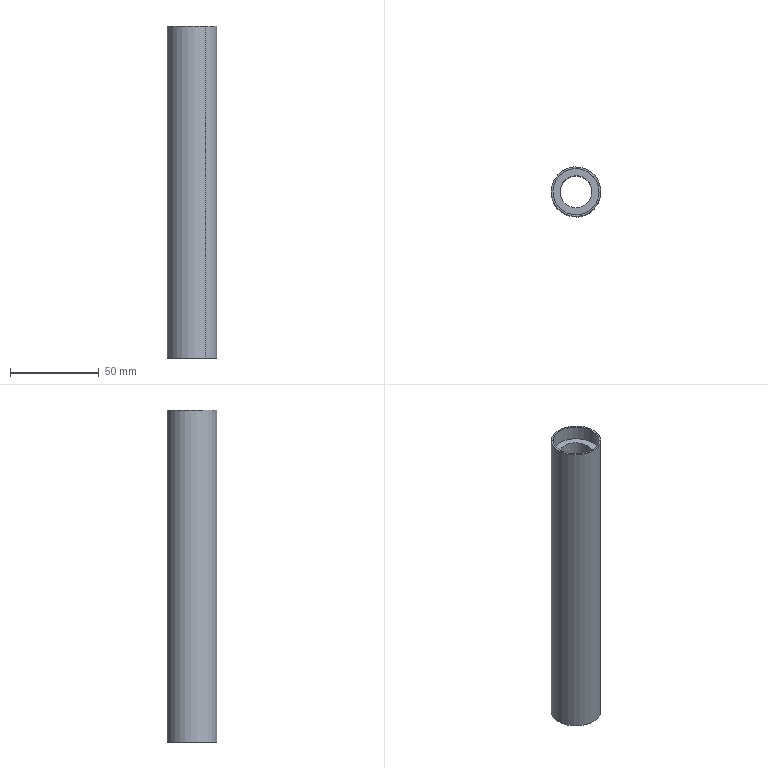Component | SolidWorks | Roller2-1 | 1 solid | 12 faces | box 28 x 28 x 187 mm | volume 63137 mm3 | cylinder 8 | plane 4 | commonest cylinder face diameters 26 x4 18 x2 28 x2
build123d program:
from build123d import *

# Parameters (mm, degrees)
MOVE_FACE1_BY = 1


with BuildPart() as part:
    # Sketch1 → Revolve1 (revolve)
    with BuildSketch(Plane(origin=(0, 0, 0), x_dir=(-1, 0, 0), z_dir=(0, 0, -1)), mode=Mode.PRIVATE) as revolve1_sk:
        Polygon((-85.5, 13), (-85.5, 9), (85.5, 9), (85.5, 13), (93.5, 13), (93.5, 15), (-93.5, 15), (-93.5, 13), align=None)
    revolve(revolve1_sk.sketch.rotate(Axis((93.5, 0, 0), (-1, 0, 0)), 270), axis=Axis((93.5, 0, 0), (-1, 0, 0)))

    # Move Face1: a curved face moved inward by 1.0
    add(Solid.thicken(part.faces().sort_by_distance((0, 0, -15))[0], -MOVE_FACE1_BY), mode=Mode.SUBTRACT)


solid = part.part

# Placed as in the assembly
solid = solid.moved(Location((-66, -158, -96.5), (0, 90, 0)))
STEP:
#1=COLOUR_RGB('',0.7922,0.8196,0.9333);
#2=FILL_AREA_STYLE_COLOUR('',#1);
#3=FILL_AREA_STYLE('',(#2));
#4=SURFACE_STYLE_FILL_AREA(#3);
#5=SURFACE_SIDE_STYLE('',(#4));
#6=SURFACE_STYLE_USAGE(.BOTH.,#5);
#7=PRESENTATION_STYLE_ASSIGNMENT((#6));
#8=CARTESIAN_POINT('',(-2.407,-6.519,-0.4331));
#9=VERTEX_POINT('',#8);
#10=CARTESIAN_POINT('',(-2.79,-5.922,-0.4331));
#11=VERTEX_POINT('',#10);
#12=CARTESIAN_POINT('',(-2.598,-6.22,-0.4331));
#13=DIRECTION('',(-0.,0.,-1.));
#14=DIRECTION('',(-0.5401,0.8416,0.));
#15=AXIS2_PLACEMENT_3D('',#12,#13,#14);
#16=CIRCLE('',#15,0.3543);
#17=EDGE_CURVE('',#9,#11,#16,.T.);
#18=ORIENTED_EDGE('',*,*,#17,.F.);
#19=CARTESIAN_POINT('',(-2.407,-6.519,-7.165));
#20=VERTEX_POINT('',#19);
#21=CARTESIAN_POINT('',(-2.407,-6.519,-0.1181));
#22=DIRECTION('',(-0.,0.,-1.));
#23=VECTOR('',#22,39.37);
#24=LINE('',#21,#23);
#25=EDGE_CURVE('',#9,#20,#24,.T.);
#26=ORIENTED_EDGE('',*,*,#25,.T.);
#27=CARTESIAN_POINT('',(-2.79,-5.922,-7.165));
#28=VERTEX_POINT('',#27);
#29=CARTESIAN_POINT('',(-2.598,-6.22,-7.165));
#30=DIRECTION('',(-0.,0.,-1.));
#31=DIRECTION('',(-0.5401,0.8416,0.));
#32=AXIS2_PLACEMENT_3D('',#29,#30,#31);
#33=CIRCLE('',#32,0.3543);
#34=EDGE_CURVE('',#20,#28,#33,.T.);
#35=ORIENTED_EDGE('',*,*,#34,.T.);
#36=CARTESIAN_POINT('',(-2.79,-5.922,-0.1181));
#37=DIRECTION('',(-0.,0.,-1.));
#38=VECTOR('',#37,39.37);
#39=LINE('',#36,#38);
#40=EDGE_CURVE('',#11,#28,#39,.T.);
#41=ORIENTED_EDGE('',*,*,#40,.F.);
#42=EDGE_LOOP('',(#18,#26,#35,#41));
#43=FACE_OUTER_BOUND('',#42,.T.);
#44=CARTESIAN_POINT('',(-2.598,-6.22,-0.1181));
#45=DIRECTION('',(-0.,0.,-1.));
#46=DIRECTION('',(-0.5401,0.8416,0.));
#47=AXIS2_PLACEMENT_3D('',#44,#45,#46);
#48=CYLINDRICAL_SURFACE('',#47,0.3543);
#49=ADVANCED_FACE('',(#43),#48,.F.);
#50=CARTESIAN_POINT('',(-2.322,-6.651,-7.165));
#51=VERTEX_POINT('',#50);
#52=CARTESIAN_POINT('',(-2.875,-5.79,-7.165));
#53=VERTEX_POINT('',#52);
#54=CARTESIAN_POINT('',(-2.598,-6.22,-7.165));
#55=DIRECTION('',(-0.,0.,-1.));
#56=DIRECTION('',(-0.5401,0.8416,0.));
#57=AXIS2_PLACEMENT_3D('',#54,#55,#56);
#58=CIRCLE('',#57,0.5118);
#59=EDGE_CURVE('',#51,#53,#58,.T.);
#60=ORIENTED_EDGE('',*,*,#59,.F.);
#61=CARTESIAN_POINT('',(-2.322,-6.651,-7.48));
#62=VERTEX_POINT('',#61);
#63=CARTESIAN_POINT('',(-2.322,-6.651,-0.1181));
#64=DIRECTION('',(-0.,0.,-1.));
#65=VECTOR('',#64,39.37);
#66=LINE('',#63,#65);
#67=EDGE_CURVE('',#51,#62,#66,.T.);
#68=ORIENTED_EDGE('',*,*,#67,.T.);
#69=CARTESIAN_POINT('',(-2.875,-5.79,-7.48));
#70=VERTEX_POINT('',#69);
#71=CARTESIAN_POINT('',(-2.598,-6.22,-7.48));
#72=DIRECTION('',(-0.,0.,-1.));
#73=DIRECTION('',(-0.5401,0.8416,0.));
#74=AXIS2_PLACEMENT_3D('',#71,#72,#73);
#75=CIRCLE('',#74,0.5118);
#76=EDGE_CURVE('',#62,#70,#75,.T.);
#77=ORIENTED_EDGE('',*,*,#76,.T.);
#78=CARTESIAN_POINT('',(-2.875,-5.79,-0.1181));
#79=DIRECTION('',(-0.,0.,-1.));
#80=VECTOR('',#79,39.37);
#81=LINE('',#78,#80);
#82=EDGE_CURVE('',#53,#70,#81,.T.);
#83=ORIENTED_EDGE('',*,*,#82,.F.);
#84=EDGE_LOOP('',(#60,#68,#77,#83));
#85=FACE_OUTER_BOUND('',#84,.T.);
#86=CARTESIAN_POINT('',(-2.598,-6.22,-0.1181));
#87=DIRECTION('',(-0.,0.,-1.));
#88=DIRECTION('',(-0.5401,0.8416,0.));
#89=AXIS2_PLACEMENT_3D('',#86,#87,#88);
#90=CYLINDRICAL_SURFACE('',#89,0.5118);
#91=ADVANCED_FACE('',(#85),#90,.F.);
#92=CARTESIAN_POINT('',(-2.896,-5.757,-0.1181));
#93=VERTEX_POINT('',#92);
#94=CARTESIAN_POINT('',(-2.301,-6.684,-0.1181));
#95=VERTEX_POINT('',#94);
#96=CARTESIAN_POINT('',(-2.598,-6.22,-0.1181));
#97=DIRECTION('',(-0.,0.,-1.));
#98=DIRECTION('',(0.5401,-0.8416,-0.));
#99=AXIS2_PLACEMENT_3D('',#96,#97,#98);
#100=CIRCLE('',#99,0.5512);
#101=EDGE_CURVE('',#93,#95,#100,.T.);
#102=ORIENTED_EDGE('',*,*,#101,.T.);
#103=CARTESIAN_POINT('',(-2.301,-6.684,-7.48));
#104=VERTEX_POINT('',#103);
#105=CARTESIAN_POINT('',(-2.301,-6.684,-0.1181));
#106=DIRECTION('',(-0.,0.,-1.));
#107=VECTOR('',#106,39.37);
#108=LINE('',#105,#107);
#109=EDGE_CURVE('',#95,#104,#108,.T.);
#110=ORIENTED_EDGE('',*,*,#109,.T.);
#111=CARTESIAN_POINT('',(-2.896,-5.757,-7.48));
#112=VERTEX_POINT('',#111);
#113=CARTESIAN_POINT('',(-2.598,-6.22,-7.48));
#114=DIRECTION('',(-0.,0.,-1.));
#115=DIRECTION('',(-0.5401,0.8416,0.));
#116=AXIS2_PLACEMENT_3D('',#113,#114,#115);
#117=CIRCLE('',#116,0.5512);
#118=EDGE_CURVE('',#112,#104,#117,.T.);
#119=ORIENTED_EDGE('',*,*,#118,.F.);
#120=CARTESIAN_POINT('',(-2.896,-5.757,-0.1181));
#121=DIRECTION('',(-0.,0.,-1.));
#122=VECTOR('',#121,39.37);
#123=LINE('',#120,#122);
#124=EDGE_CURVE('',#93,#112,#123,.T.);
#125=ORIENTED_EDGE('',*,*,#124,.F.);
#126=EDGE_LOOP('',(#102,#110,#119,#125));
#127=FACE_OUTER_BOUND('',#126,.T.);
#128=CARTESIAN_POINT('',(-2.598,-6.22,-0.1181));
#129=DIRECTION('',(-0.,0.,-1.));
#130=DIRECTION('',(-0.5401,0.8416,0.));
#131=AXIS2_PLACEMENT_3D('',#128,#129,#130);
#132=CYLINDRICAL_SURFACE('',#131,0.5512);
#133=ADVANCED_FACE('',(#127),#132,.T.);
#134=CARTESIAN_POINT('',(-2.322,-6.651,-0.1181));
#135=VERTEX_POINT('',#134);
#136=CARTESIAN_POINT('',(-2.875,-5.79,-0.1181));
#137=VERTEX_POINT('',#136);
#138=CARTESIAN_POINT('',(-2.598,-6.22,-0.1181));
#139=DIRECTION('',(-0.,0.,-1.));
#140=DIRECTION('',(-0.5401,0.8416,0.));
#141=AXIS2_PLACEMENT_3D('',#138,#139,#140);
#142=CIRCLE('',#141,0.5118);
#143=EDGE_CURVE('',#135,#137,#142,.T.);
#144=ORIENTED_EDGE('',*,*,#143,.F.);
#145=CARTESIAN_POINT('',(-2.322,-6.651,-0.4331));
#146=VERTEX_POINT('',#145);
#147=CARTESIAN_POINT('',(-2.322,-6.651,-0.1181));
#148=DIRECTION('',(-0.,0.,-1.));
#149=VECTOR('',#148,39.37);
#150=LINE('',#147,#149);
#151=EDGE_CURVE('',#135,#146,#150,.T.);
#152=ORIENTED_EDGE('',*,*,#151,.T.);
#153=CARTESIAN_POINT('',(-2.875,-5.79,-0.4331));
#154=VERTEX_POINT('',#153);
#155=CARTESIAN_POINT('',(-2.598,-6.22,-0.4331));
#156=DIRECTION('',(-0.,0.,-1.));
#157=DIRECTION('',(-0.5401,0.8416,0.));
#158=AXIS2_PLACEMENT_3D('',#155,#156,#157);
#159=CIRCLE('',#158,0.5118);
#160=EDGE_CURVE('',#146,#154,#159,.T.);
#161=ORIENTED_EDGE('',*,*,#160,.T.);
#162=CARTESIAN_POINT('',(-2.875,-5.79,-0.1181));
#163=DIRECTION('',(-0.,0.,-1.));
#164=VECTOR('',#163,39.37);
#165=LINE('',#162,#164);
#166=EDGE_CURVE('',#137,#154,#165,.T.);
#167=ORIENTED_EDGE('',*,*,#166,.F.);
#168=EDGE_LOOP('',(#144,#152,#161,#167));
#169=FACE_OUTER_BOUND('',#168,.T.);
#170=CARTESIAN_POINT('',(-2.598,-6.22,-0.1181));
#171=DIRECTION('',(-0.,0.,-1.));
#172=DIRECTION('',(-0.5401,0.8416,0.));
#173=AXIS2_PLACEMENT_3D('',#170,#171,#172);
#174=CYLINDRICAL_SURFACE('',#173,0.5118);
#175=ADVANCED_FACE('',(#169),#174,.F.);
#176=ORIENTED_EDGE('',*,*,#151,.F.);
#177=CARTESIAN_POINT('',(-2.598,-6.22,-0.1181));
#178=DIRECTION('',(-0.,0.,-1.));
#179=DIRECTION('',(-0.5401,0.8416,0.));
#180=AXIS2_PLACEMENT_3D('',#177,#178,#179);
#181=CIRCLE('',#180,0.5118);
#182=EDGE_CURVE('',#137,#135,#181,.T.);
#183=ORIENTED_EDGE('',*,*,#182,.F.);
#184=ORIENTED_EDGE('',*,*,#166,.T.);
#185=CARTESIAN_POINT('',(-2.598,-6.22,-0.4331));
#186=DIRECTION('',(-0.,0.,-1.));
#187=DIRECTION('',(-0.5401,0.8416,0.));
#188=AXIS2_PLACEMENT_3D('',#185,#186,#187);
#189=CIRCLE('',#188,0.5118);
#190=EDGE_CURVE('',#154,#146,#189,.T.);
#191=ORIENTED_EDGE('',*,*,#190,.T.);
#192=EDGE_LOOP('',(#176,#183,#184,#191));
#193=FACE_OUTER_BOUND('',#192,.T.);
#194=CARTESIAN_POINT('',(-2.598,-6.22,-0.1181));
#195=DIRECTION('',(-0.,0.,-1.));
#196=DIRECTION('',(-0.5401,0.8416,0.));
#197=AXIS2_PLACEMENT_3D('',#194,#195,#196);
#198=CYLINDRICAL_SURFACE('',#197,0.5118);
#199=ADVANCED_FACE('',(#193),#198,.F.);
#200=ORIENTED_EDGE('',*,*,#182,.T.);
#201=ORIENTED_EDGE('',*,*,#143,.T.);
#202=EDGE_LOOP('',(#200,#201));
#203=FACE_BOUND('',#202,.T.);
#204=ORIENTED_EDGE('',*,*,#101,.F.);
#205=CARTESIAN_POINT('',(-2.598,-6.22,-0.1181));
#206=DIRECTION('',(-0.,0.,-1.));
#207=DIRECTION('',(0.5401,-0.8416,-0.));
#208=AXIS2_PLACEMENT_3D('',#205,#206,#207);
#209=CIRCLE('',#208,0.5512);
#210=EDGE_CURVE('',#95,#93,#209,.T.);
#211=ORIENTED_EDGE('',*,*,#210,.F.);
#212=EDGE_LOOP('',(#204,#211));
#213=FACE_OUTER_BOUND('',#212,.T.);
#214=CARTESIAN_POINT('',(-2.101,-5.902,-0.1181));
#215=DIRECTION('',(0.,-0.,1.));
#216=DIRECTION('',(0.5401,-0.8416,-0.));
#217=AXIS2_PLACEMENT_3D('',#214,#215,#216);
#218=PLANE('',#217);
#219=ADVANCED_FACE('',(#203,#213),#218,.T.);
#220=ORIENTED_EDGE('',*,*,#109,.F.);
#221=ORIENTED_EDGE('',*,*,#210,.T.);
#222=ORIENTED_EDGE('',*,*,#124,.T.);
#223=CARTESIAN_POINT('',(-2.598,-6.22,-7.48));
#224=DIRECTION('',(-0.,0.,-1.));
#225=DIRECTION('',(-0.5401,0.8416,0.));
#226=AXIS2_PLACEMENT_3D('',#223,#224,#225);
#227=CIRCLE('',#226,0.5512);
#228=EDGE_CURVE('',#104,#112,#227,.T.);
#229=ORIENTED_EDGE('',*,*,#228,.F.);
#230=EDGE_LOOP('',(#220,#221,#222,#229));
#231=FACE_OUTER_BOUND('',#230,.T.);
#232=CARTESIAN_POINT('',(-2.598,-6.22,-0.1181));
#233=DIRECTION('',(-0.,0.,-1.));
#234=DIRECTION('',(-0.5401,0.8416,0.));
#235=AXIS2_PLACEMENT_3D('',#232,#233,#234);
#236=CYLINDRICAL_SURFACE('',#235,0.5512);
#237=ADVANCED_FACE('',(#231),#236,.T.);
#238=ORIENTED_EDGE('',*,*,#118,.T.);
#239=ORIENTED_EDGE('',*,*,#228,.T.);
#240=EDGE_LOOP('',(#238,#239));
#241=FACE_OUTER_BOUND('',#240,.T.);
#242=CARTESIAN_POINT('',(-2.598,-6.22,-7.48));
#243=DIRECTION('',(-0.,0.,-1.));
#244=DIRECTION('',(-0.5401,0.8416,0.));
#245=AXIS2_PLACEMENT_3D('',#242,#243,#244);
#246=CIRCLE('',#245,0.5118);
#247=EDGE_CURVE('',#70,#62,#246,.T.);
#248=ORIENTED_EDGE('',*,*,#247,.F.);
#249=ORIENTED_EDGE('',*,*,#76,.F.);
#250=EDGE_LOOP('',(#248,#249));
#251=FACE_BOUND('',#250,.T.);
#252=CARTESIAN_POINT('',(-2.168,-5.944,-7.48));
#253=DIRECTION('',(-0.,0.,-1.));
#254=DIRECTION('',(-0.5401,0.8416,0.));
#255=AXIS2_PLACEMENT_3D('',#252,#253,#254);
#256=PLANE('',#255);
#257=ADVANCED_FACE('',(#241,#251),#256,.T.);
#258=ORIENTED_EDGE('',*,*,#67,.F.);
#259=CARTESIAN_POINT('',(-2.598,-6.22,-7.165));
#260=DIRECTION('',(-0.,0.,-1.));
#261=DIRECTION('',(-0.5401,0.8416,0.));
#262=AXIS2_PLACEMENT_3D('',#259,#260,#261);
#263=CIRCLE('',#262,0.5118);
#264=EDGE_CURVE('',#53,#51,#263,.T.);
#265=ORIENTED_EDGE('',*,*,#264,.F.);
#266=ORIENTED_EDGE('',*,*,#82,.T.);
#267=ORIENTED_EDGE('',*,*,#247,.T.);
#268=EDGE_LOOP('',(#258,#265,#266,#267));
#269=FACE_OUTER_BOUND('',#268,.T.);
#270=CARTESIAN_POINT('',(-2.598,-6.22,-0.1181));
#271=DIRECTION('',(-0.,0.,-1.));
#272=DIRECTION('',(-0.5401,0.8416,0.));
#273=AXIS2_PLACEMENT_3D('',#270,#271,#272);
#274=CYLINDRICAL_SURFACE('',#273,0.5118);
#275=ADVANCED_FACE('',(#269),#274,.F.);
#276=ORIENTED_EDGE('',*,*,#264,.T.);
#277=ORIENTED_EDGE('',*,*,#59,.T.);
#278=EDGE_LOOP('',(#276,#277));
#279=FACE_OUTER_BOUND('',#278,.T.);
#280=CARTESIAN_POINT('',(-2.598,-6.22,-7.165));
#281=DIRECTION('',(-0.,0.,-1.));
#282=DIRECTION('',(-0.5401,0.8416,0.));
#283=AXIS2_PLACEMENT_3D('',#280,#281,#282);
#284=CIRCLE('',#283,0.3543);
#285=EDGE_CURVE('',#28,#20,#284,.T.);
#286=ORIENTED_EDGE('',*,*,#285,.F.);
#287=ORIENTED_EDGE('',*,*,#34,.F.);
#288=EDGE_LOOP('',(#286,#287));
#289=FACE_BOUND('',#288,.T.);
#290=CARTESIAN_POINT('',(-2.3,-6.029,-7.165));
#291=DIRECTION('',(-0.,0.,-1.));
#292=DIRECTION('',(-0.5401,0.8416,0.));
#293=AXIS2_PLACEMENT_3D('',#290,#291,#292);
#294=PLANE('',#293);
#295=ADVANCED_FACE('',(#279,#289),#294,.T.);
#296=ORIENTED_EDGE('',*,*,#25,.F.);
#297=CARTESIAN_POINT('',(-2.598,-6.22,-0.4331));
#298=DIRECTION('',(-0.,0.,-1.));
#299=DIRECTION('',(-0.5401,0.8416,0.));
#300=AXIS2_PLACEMENT_3D('',#297,#298,#299);
#301=CIRCLE('',#300,0.3543);
#302=EDGE_CURVE('',#11,#9,#301,.T.);
#303=ORIENTED_EDGE('',*,*,#302,.F.);
#304=ORIENTED_EDGE('',*,*,#40,.T.);
#305=ORIENTED_EDGE('',*,*,#285,.T.);
#306=EDGE_LOOP('',(#296,#303,#304,#305));
#307=FACE_OUTER_BOUND('',#306,.T.);
#308=CARTESIAN_POINT('',(-2.598,-6.22,-0.1181));
#309=DIRECTION('',(-0.,0.,-1.));
#310=DIRECTION('',(-0.5401,0.8416,0.));
#311=AXIS2_PLACEMENT_3D('',#308,#309,#310);
#312=CYLINDRICAL_SURFACE('',#311,0.3543);
#313=ADVANCED_FACE('',(#307),#312,.F.);
#314=ORIENTED_EDGE('',*,*,#302,.T.);
#315=ORIENTED_EDGE('',*,*,#17,.T.);
#316=EDGE_LOOP('',(#314,#315));
#317=FACE_BOUND('',#316,.T.);
#318=ORIENTED_EDGE('',*,*,#190,.F.);
#319=ORIENTED_EDGE('',*,*,#160,.F.);
#320=EDGE_LOOP('',(#318,#319));
#321=FACE_OUTER_BOUND('',#320,.T.);
#322=CARTESIAN_POINT('',(-2.168,-5.944,-0.4331));
#323=DIRECTION('',(0.,-0.,1.));
#324=DIRECTION('',(0.5401,-0.8416,-0.));
#325=AXIS2_PLACEMENT_3D('',#322,#323,#324);
#326=PLANE('',#325);
#327=ADVANCED_FACE('',(#317,#321),#326,.T.);
#328=CLOSED_SHELL('',(#49,#91,#133,#175,#199,#219,#237,#257,#275,#295,#313,#327));
#329=MANIFOLD_SOLID_BREP('',#328);
#330=STYLED_ITEM('',(#7),#329);
#331=(LENGTH_UNIT()NAMED_UNIT(*)SI_UNIT($,.METRE.));
#332=LENGTH_MEASURE_WITH_UNIT(LENGTH_MEASURE(0.0254),#331);
#333=DIMENSIONAL_EXPONENTS(1.,0.,0.,0.,0.,0.,0.);
#334=(CONVERSION_BASED_UNIT('',#332)LENGTH_UNIT()NAMED_UNIT(#333));
#335=UNCERTAINTY_MEASURE_WITH_UNIT(LENGTH_MEASURE(0.00001),#334,'','');
#336=(NAMED_UNIT(*)PLANE_ANGLE_UNIT()SI_UNIT($,.RADIAN.));
#337=(NAMED_UNIT(*)SI_UNIT($,.STERADIAN.)SOLID_ANGLE_UNIT());
#338=(GEOMETRIC_REPRESENTATION_CONTEXT(3)GLOBAL_UNCERTAINTY_ASSIGNED_CONTEXT((#335))GLOBAL_UNIT_ASSIGNED_CONTEXT((#334,#336,#337))REPRESENTATION_CONTEXT('',''));
#339=MECHANICAL_DESIGN_GEOMETRIC_PRESENTATION_REPRESENTATION('',(#330),#338);
#340=CARTESIAN_POINT('',(0.,0.,0.));
#341=DIRECTION('',(0.,0.,1.));
#342=DIRECTION('',(1.,0.,0.));
#343=AXIS2_PLACEMENT_3D('',#340,#341,#342);
#344=(LENGTH_UNIT()NAMED_UNIT(*)SI_UNIT($,.METRE.));
#345=LENGTH_MEASURE_WITH_UNIT(LENGTH_MEASURE(0.0254),#344);
#346=DIMENSIONAL_EXPONENTS(1.,0.,0.,0.,0.,0.,0.);
#347=(CONVERSION_BASED_UNIT('',#345)LENGTH_UNIT()NAMED_UNIT(#346));
#348=UNCERTAINTY_MEASURE_WITH_UNIT(LENGTH_MEASURE(0.00001),#347,'','');
#349=(NAMED_UNIT(*)PLANE_ANGLE_UNIT()SI_UNIT($,.RADIAN.));
#350=(NAMED_UNIT(*)SI_UNIT($,.STERADIAN.)SOLID_ANGLE_UNIT());
#351=(GEOMETRIC_REPRESENTATION_CONTEXT(3)GLOBAL_UNCERTAINTY_ASSIGNED_CONTEXT((#348))GLOBAL_UNIT_ASSIGNED_CONTEXT((#347,#349,#350))REPRESENTATION_CONTEXT('',''));
#352=ADVANCED_BREP_SHAPE_REPRESENTATION('',(#329,#343),#351);
#353=PRESENTATION_LAYER_ASSIGNMENT('','',(#330));